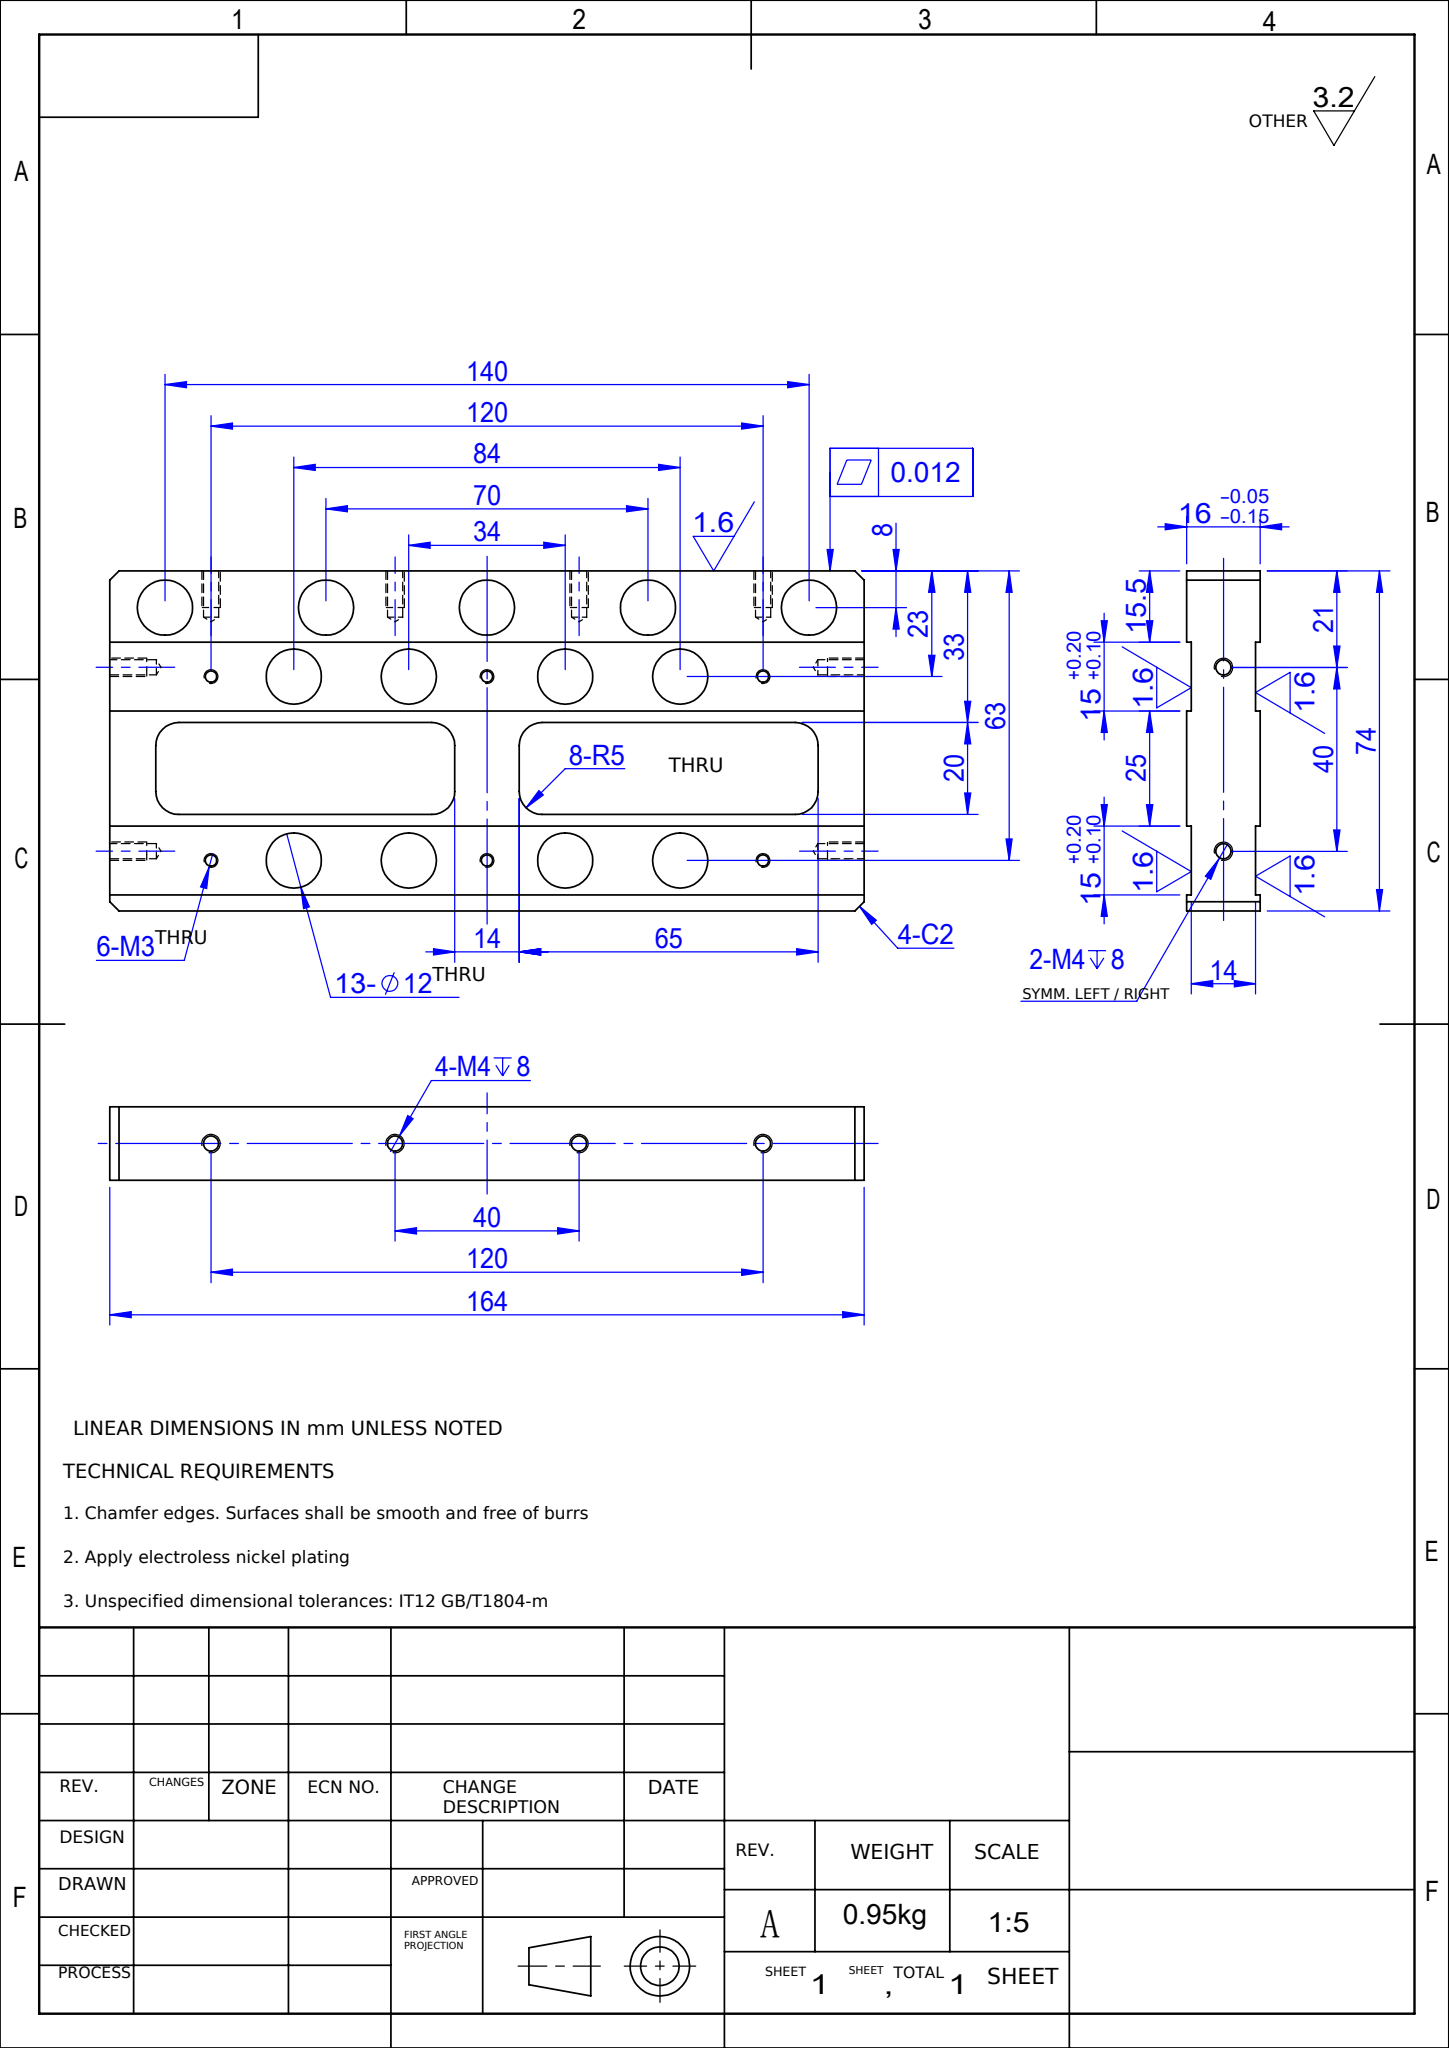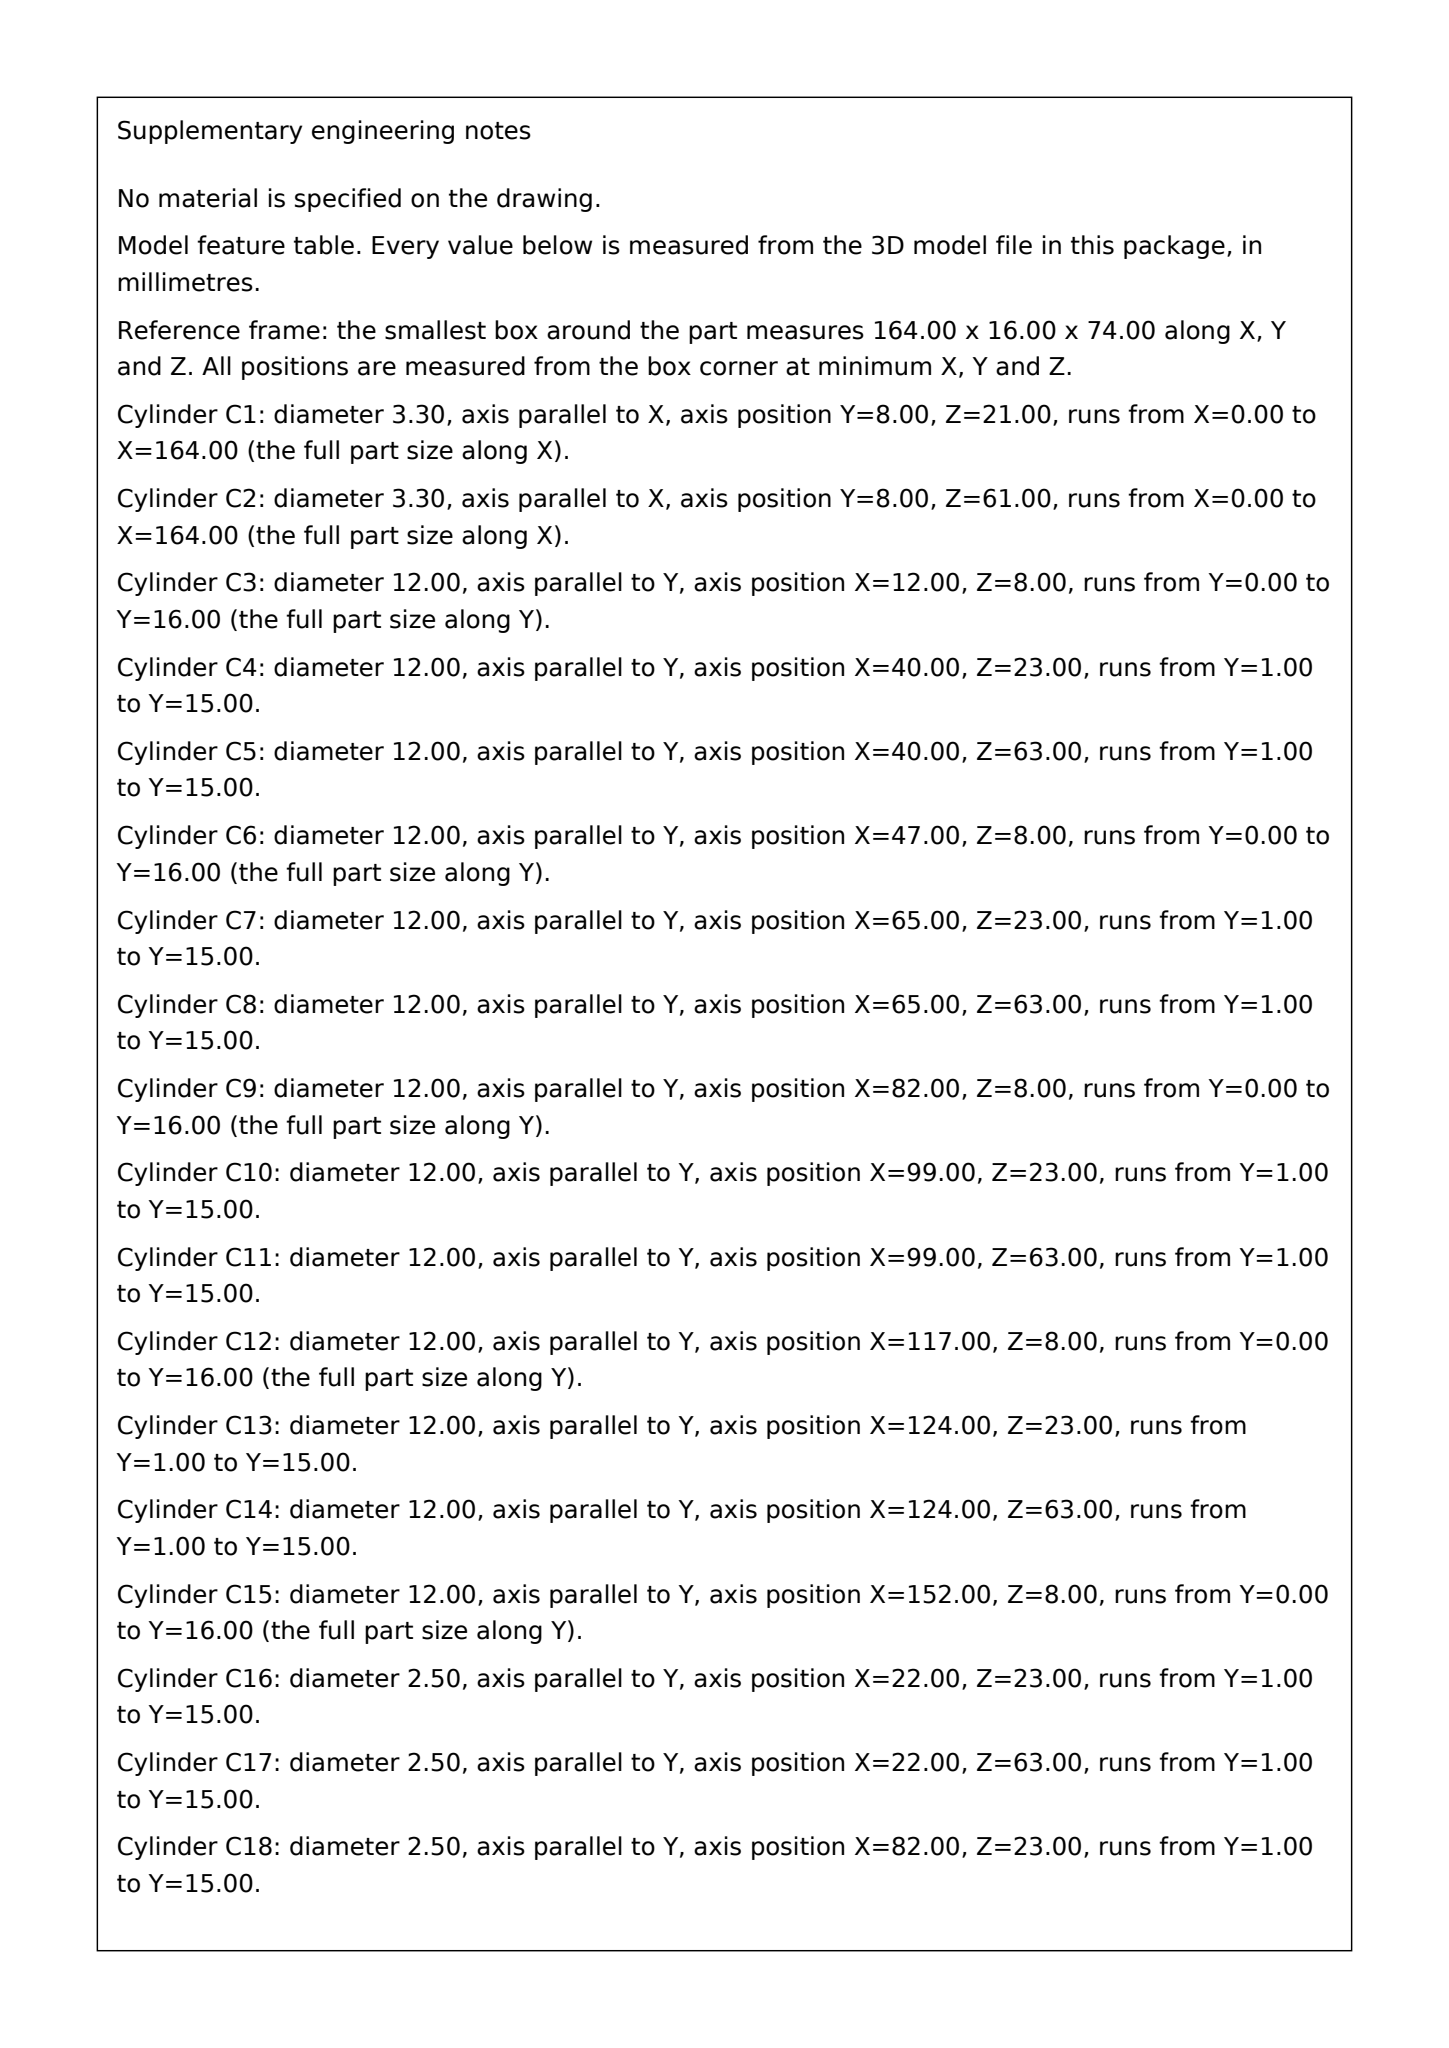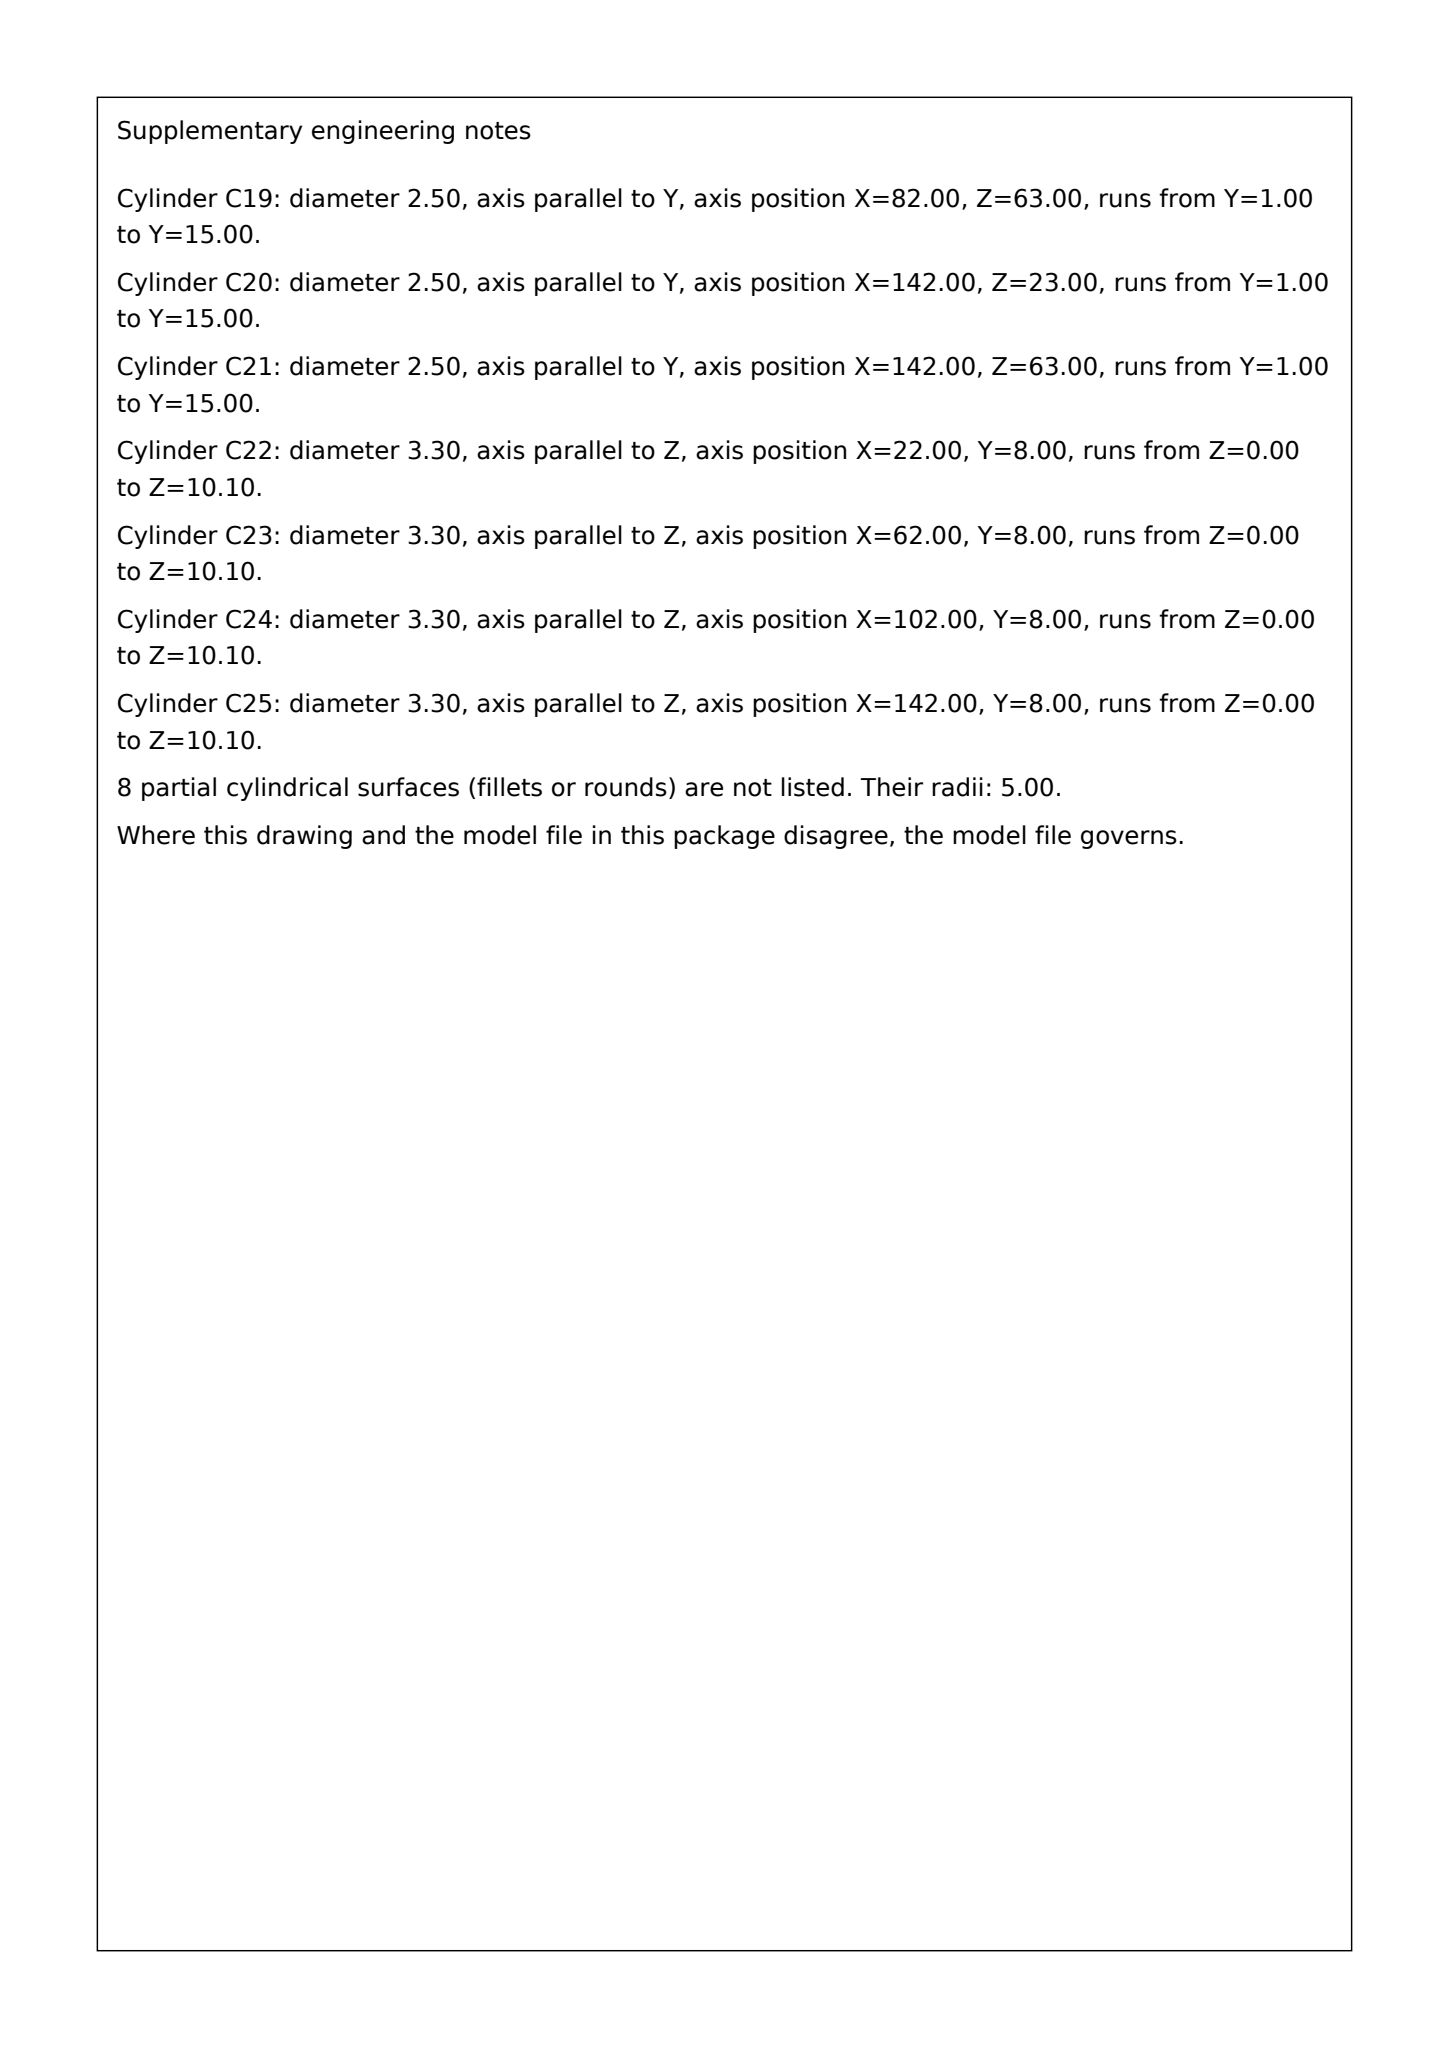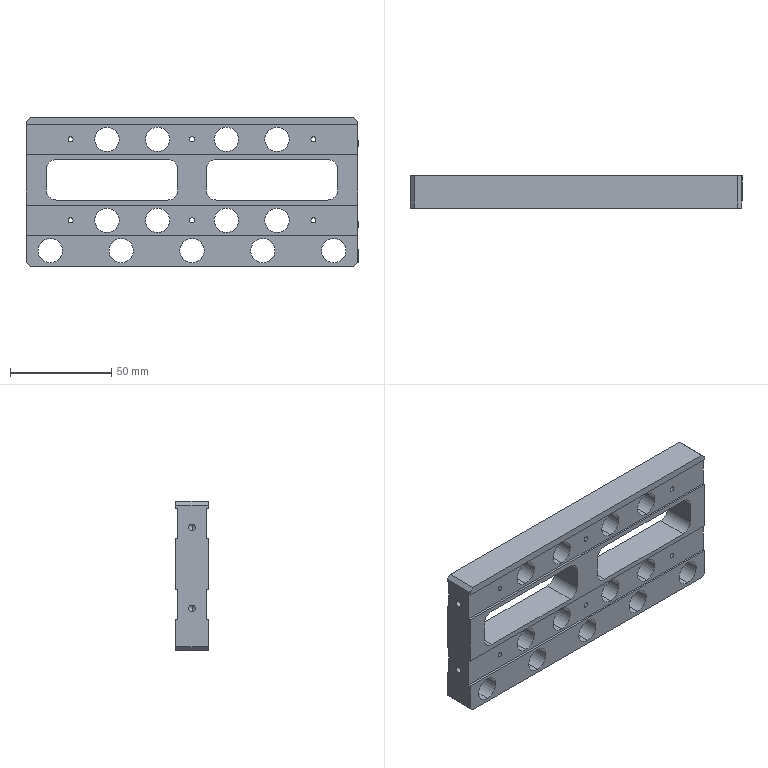Part | SolidWorks | mm | material Q235-A | 1 solid | 112 faces | box 164 x 16 x 74 mm | volume 120454 mm3 | cylinder 62 | plane 34 | cone 16 | commonest cylinder face diameters 12 x26 3.3 x16 2.5 x12 10 x8
build123d program:
from build123d import *

# Parameters (mm, degrees)
SKETCH1_W                  = 164
SKETCH1_H                  = 74
BOSS_EXTRUDE1_DEPTH        = 8
SKETCH2_W                  = 15
SKETCH2_H                  = 1
CUT_EXTRUDE1_DEPTH         = 169.312
CHAMFER1_SIZE              = 2
M3_TAPPED_HOLE1_D          = 2.5
LPATTERN1_COUNT            = 3
LPATTERN1_PITCH            = 60
LPATTERN1_COUNT_DIR2       = 2
LPATTERN1_PITCH_DIR2       = 40
F_12_0_12_DIAMETER_HOLE1_D = 12
LPATTERN2_COUNT            = 2
LPATTERN2_PITCH            = 25
LPATTERN3_COUNT            = 4
LPATTERN3_PITCH            = 40
M4_TAPPED_HOLE2_AT_2_COUNT = 2
M4_TAPPED_HOLE2_AT_2_PITCH = 40
MIRROR3_COPY_1_D           = 12
LPATTERN4_COUNT            = 2
LPATTERN4_PITCH            = 40
LPATTERN4_COPY_1_D         = 12
LPATTERN4_COPY_2_D         = 12
LPATTERN4_COPY_3_D         = 12
SKETCH11_W                 = 65
SKETCH11_H                 = 20
CUT_EXTRUDE2_DEPTH         = 92.373
FILLET1_R                  = 5
FILLET1_OF_MIRROR4_R       = 5
F_12_0_12_DIAMETER_HOLE2_D = 12
LPATTERN5_COUNT            = 5
LPATTERN5_PITCH            = 35


with BuildPart() as part:
    # Sketch1 → Boss-Extrude1 (new, symmetric)
    with BuildSketch(Plane(origin=(0, 0, 0), x_dir=(1, 0, 0), z_dir=(0, 1, 0))):
        Rectangle(SKETCH1_W, SKETCH1_H)
    extrude(amount=BOSS_EXTRUDE1_DEPTH, both=True)

    # Sketch2 → Cut-Extrude1 (cut, through all)
    with BuildSketch(Plane(origin=(82, 0, 0), x_dir=(0, 0, -1), z_dir=(1, 0, 0))):
        with Locations((14, 7.5)):
            Rectangle(SKETCH2_W, SKETCH2_H)
        with Locations((-26, 7.5)):
            Rectangle(SKETCH2_W, SKETCH2_H)
    cut_extrude1 = extrude(amount=-CUT_EXTRUDE1_DEPTH, mode=Mode.SUBTRACT)

    # Mirror1: Cut-Extrude1 across plane
    add(cut_extrude1.mirror(Plane.ZX), mode=Mode.SUBTRACT)

    # Chamfer1
    chamfer1_edges = [part.edges().sort_by_distance(p)[0] for p in [
        (-82, 0, -37),
        (82, 0, -37),
        (82, 0, 37),
        (-82, 0, 37),
    ]]
    chamfer(chamfer1_edges, length=CHAMFER1_SIZE)

    # M3 Tapped Hole1 (through all)
    with Locations(Plane(origin=(0, 7, 0), x_dir=(-1, 0, 0), z_dir=(0, 1, 0))):
        with Locations((-60, -14)):
            m3_tapped_hole1 = Hole(M3_TAPPED_HOLE1_D / 2)

    # LPattern1: M3 Tapped Hole1 3 × 2
    with Locations(*[(-i * LPATTERN1_PITCH, 0, j * LPATTERN1_PITCH_DIR2) for i in range(LPATTERN1_COUNT) for j in range(LPATTERN1_COUNT_DIR2) if (i, j) != (0, 0)]):
        add(m3_tapped_hole1, mode=Mode.SUBTRACT)

    # 12.0 _12_ Diameter Hole1 (through all)
    with Locations(Plane(origin=(0, 8, 0), x_dir=(-1, 0, 0), z_dir=(0, 1, 0))):
        with Locations((-42, 26)):
            f_12_0_12_diameter_hole1 = Hole(F_12_0_12_DIAMETER_HOLE1_D / 2)

    # LPattern2: 12.0 _12_ Diameter Hole1 ×2
    with Locations(*[(-i * LPATTERN2_PITCH, 0, 0) for i in range(1, LPATTERN2_COUNT)]):
        add(f_12_0_12_diameter_hole1, mode=Mode.SUBTRACT)

    # Sketch7 → M4 Tapped Hole1 (revolve, cut)
    with BuildSketch(Plane(origin=(-60, 0, -37), x_dir=(0, 1, 0), z_dir=(1, 0, 0))):
        Polygon((0, 0), (0, 11.091), (1.65, 10.1), (1.65, 0), align=None)
    m4_tapped_hole1 = revolve(axis=Axis((-60, 0, -43.35), (0, 0, 1)), mode=Mode.SUBTRACT)

    # LPattern3: M4 Tapped Hole1 ×4
    with Locations(*[(i * LPATTERN3_PITCH, 0, 0) for i in range(1, LPATTERN3_COUNT)]):
        add(m4_tapped_hole1, mode=Mode.SUBTRACT)

    # Sketch9 → M4 Tapped Hole2 (revolve, cut)
    with BuildSketch(Plane(origin=(-82, 0, -16), x_dir=(0, 0, 1), z_dir=(0, 1, 0))):
        Polygon((0, 0), (0, 11.091), (1.65, 10.1), (1.65, 0), align=None)
    m4_tapped_hole2 = revolve(axis=Axis((-88.35, 0, -16), (1, 0, 0)), mode=Mode.SUBTRACT)

    # M4 Tapped Hole2 at 2: M4 Tapped Hole2 ×2
    with Locations(*[(0, 0, i * M4_TAPPED_HOLE2_AT_2_PITCH) for i in range(1, M4_TAPPED_HOLE2_AT_2_COUNT)]):
        add(m4_tapped_hole2, mode=Mode.SUBTRACT)

    # Mirror2: M4 Tapped Hole2 across plane
    add(m4_tapped_hole2.mirror(Plane(origin=(0, 0, 0), x_dir=(0, 0, 1), z_dir=(1, 0, 0))), mode=Mode.SUBTRACT)

    # Mirror2 copy 1 sketch → Mirror2 copy 1 (revolve, cut)
    with BuildSketch(Plane(origin=(82, 0, 24), x_dir=(0, 0, 1), z_dir=(0, 1, 0))):
        Polygon((0, 0), (0, -11.091), (1.65, -10.1), (1.65, 0), align=None)
    revolve(axis=Axis((88.35, 0, 24), (1, 0, 0)), mode=Mode.SUBTRACT)

    # Mirror3: 12.0 _12_ Diameter Hole1 across plane
    add(f_12_0_12_diameter_hole1.mirror(Plane(origin=(0, 0, 0), x_dir=(0, 0, 1), z_dir=(1, 0, 0))), mode=Mode.SUBTRACT)

    # Mirror3 copy 1 (through all)
    with Locations(Plane(origin=(25, 8, 0), x_dir=(1, 0, 0), z_dir=(0, 1, 0))):
        with Locations((-42, -26)):
            Hole(MIRROR3_COPY_1_D / 2)

    # LPattern4: 12.0 _12_ Diameter Hole1 ×2
    with Locations(*[(0, 0, -i * LPATTERN4_PITCH) for i in range(1, LPATTERN4_COUNT)]):
        add(f_12_0_12_diameter_hole1, mode=Mode.SUBTRACT)

    # LPattern4 copy 1 (through all)
    with Locations(Plane(origin=(-25, 8, -40), x_dir=(-1, 0, 0), z_dir=(0, 1, 0))):
        with Locations((-42, 26)):
            Hole(LPATTERN4_COPY_1_D / 2)

    # LPattern4 copy 2 (through all)
    with Locations(Plane(origin=(0, 8, -40), x_dir=(1, 0, 0), z_dir=(0, 1, 0))):
        with Locations((-42, -26)):
            Hole(LPATTERN4_COPY_2_D / 2)

    # LPattern4 copy 3 (through all)
    with Locations(Plane(origin=(25, 8, -40), x_dir=(1, 0, 0), z_dir=(0, 1, 0))):
        with Locations((-42, -26)):
            Hole(LPATTERN4_COPY_3_D / 2)

    # Sketch11 → Cut-Extrude2 (cut, through all)
    with BuildSketch(Plane(origin=(0, 8, 0), x_dir=(1, 0, 0), z_dir=(0, 1, 0))):
        with Locations((-39.5, -6)):
            Rectangle(SKETCH11_W, SKETCH11_H)
    cut_extrude2 = extrude(amount=-CUT_EXTRUDE2_DEPTH, mode=Mode.SUBTRACT)

    # Fillet1
    fillet1_edges = [part.edges().sort_by_distance(p)[0] for p in [
        (-72, 0, 16),
        (-72, 0, -4),
        (-7, 0, -4),
        (-7, 0, 16),
    ]]
    fillet(fillet1_edges, radius=FILLET1_R)

    # Mirror4: Cut-Extrude2 across plane
    add(cut_extrude2.mirror(Plane(origin=(0, 0, 0), x_dir=(0, 0, 1), z_dir=(1, 0, 0))), mode=Mode.SUBTRACT)

    # Fillet1 of Mirror4
    fillet1_of_mirror4_edges = [part.edges().sort_by_distance(p)[0] for p in [
        (72, 0, 16),
        (72, 0, -4),
        (7, 0, -4),
        (7, 0, 16),
    ]]
    fillet(fillet1_of_mirror4_edges, radius=FILLET1_OF_MIRROR4_R)

    # 12.0 _12_ Diameter Hole2 (through all)
    with Locations(Plane(origin=(0, 8, 0), x_dir=(-1, 0, 0), z_dir=(0, 1, 0))):
        with Locations((-70, -29)):
            f_12_0_12_diameter_hole2 = Hole(F_12_0_12_DIAMETER_HOLE2_D / 2)

    # LPattern5: 12.0 _12_ Diameter Hole2 ×5
    with Locations(*[(-i * LPATTERN5_PITCH, 0, 0) for i in range(1, LPATTERN5_COUNT)]):
        add(f_12_0_12_diameter_hole2, mode=Mode.SUBTRACT)


solid = part.part